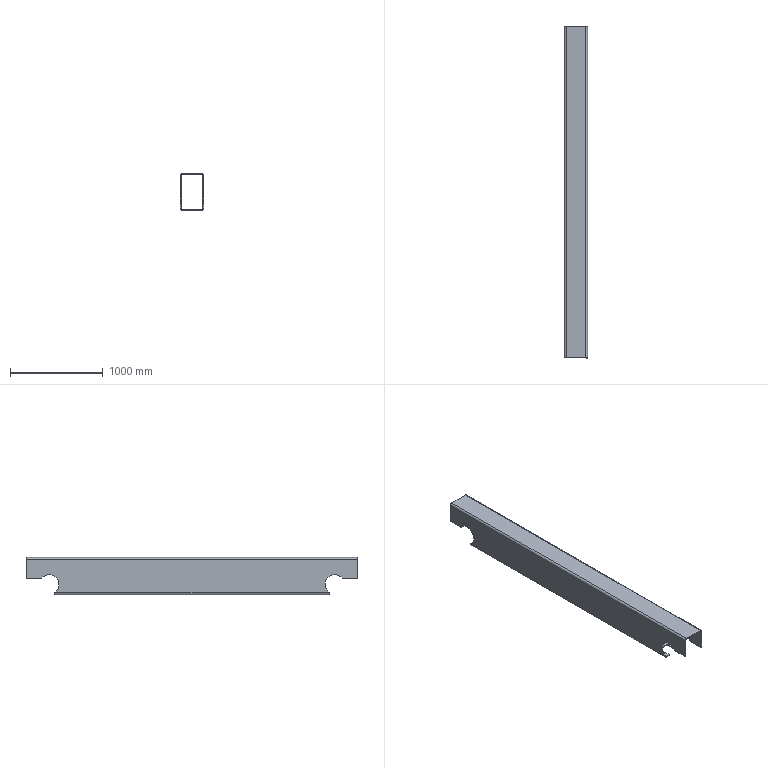Component | SolidWorks | Short-1_3650-1 | 1 solid | 46 faces | box 250 x 3580 x 400 mm | volume 39951566 mm3 | plane 24 | cylinder 22 | commonest cylinder face diameters 20 x12 210 x6 40 x4
build123d program:
from build123d import *

# Parameters (mm, degrees)
BOSS_EXTRUDE1_DEPTH = 1790
CUT_EXTRUDE1_DEPTH  = 1819.406
SKETCH2_W           = 120
SKETCH2_H           = 150
CUT_EXTRUDE2_DEPTH  = 10


with BuildPart() as part:
    # Sketch1 → Boss-Extrude1 (new, symmetric)
    with BuildSketch(Plane.XY):
        with BuildLine():
            Line((-105, -200), (105, -200))
            ThreePointArc((105, -200), (119.142, -194.142), (125, -180))
            Line((125, -180), (125, 180))
            ThreePointArc((125, 180), (119.142, 194.142), (105, 200))
            Line((105, 200), (-105, 200))
            ThreePointArc((-105, 200), (-119.142, 194.142), (-125, 180))
            Line((-125, 180), (-125, -180))
            ThreePointArc((-125, -180), (-119.142, -194.142), (-105, -200))
        make_face()
        with BuildLine():
            Line((-105, -190), (105, -190))
            ThreePointArc((105, -190), (112.071, -187.071), (115, -180))
            Line((115, -180), (115, 180))
            ThreePointArc((115, 180), (112.071, 187.071), (105, 190))
            Line((105, 190), (-105, 190))
            ThreePointArc((-105, 190), (-112.071, 187.071), (-115, 180))
            Line((-115, 180), (-115, -180))
            ThreePointArc((-115, -180), (-112.071, -187.071), (-105, -190))
        make_face(mode=Mode.SUBTRACT)
    extrude(amount=BOSS_EXTRUDE1_DEPTH, both=True)

    # Sketch1_2 → Cut-Extrude1 (cut, through all)
    with BuildSketch(Plane(origin=(125, 0, 0), x_dir=(0, 0, -1), z_dir=(1, 0, 0))):
        with BuildLine():
            Line((-1480, -200), (-1790, -200))
            Line((-1790, -200), (-1790, -30))
            Line((-1790, -30), (-1631.241, -30))
            ThreePointArc((-1631.241, -30), (-1626.818, -28.969), (-1623.307, -26.087))
            ThreePointArc((-1623.307, -26.087), (-1465.754, -15.754), (-1476.087, -173.307))
            ThreePointArc((-1476.087, -173.307), (-1478.969, -176.818), (-1480, -181.241))
            Line((-1480, -181.241), (-1480, -200))
        make_face()
    cut_extrude1 = extrude(amount=-CUT_EXTRUDE1_DEPTH, mode=Mode.SUBTRACT)

    # Sketch2 → Cut-Extrude2 (cut)
    with BuildSketch(Plane.XZ.offset(200)):
        with Locations((0, 1405)):
            Rectangle(SKETCH2_W, SKETCH2_H)
    cut_extrude2 = extrude(amount=-CUT_EXTRUDE2_DEPTH, mode=Mode.SUBTRACT)

    # Mirror1: Cut-Extrude1, Cut-Extrude2 across plane
    add(cut_extrude1.mirror(Plane.XY), mode=Mode.SUBTRACT)
    add(cut_extrude2.mirror(Plane.XY), mode=Mode.SUBTRACT)


solid = part.part

# Placed as in the assembly
solid = solid.moved(Location((-3237.199, 1171.323, 4985.973), (90, 0, 0)))